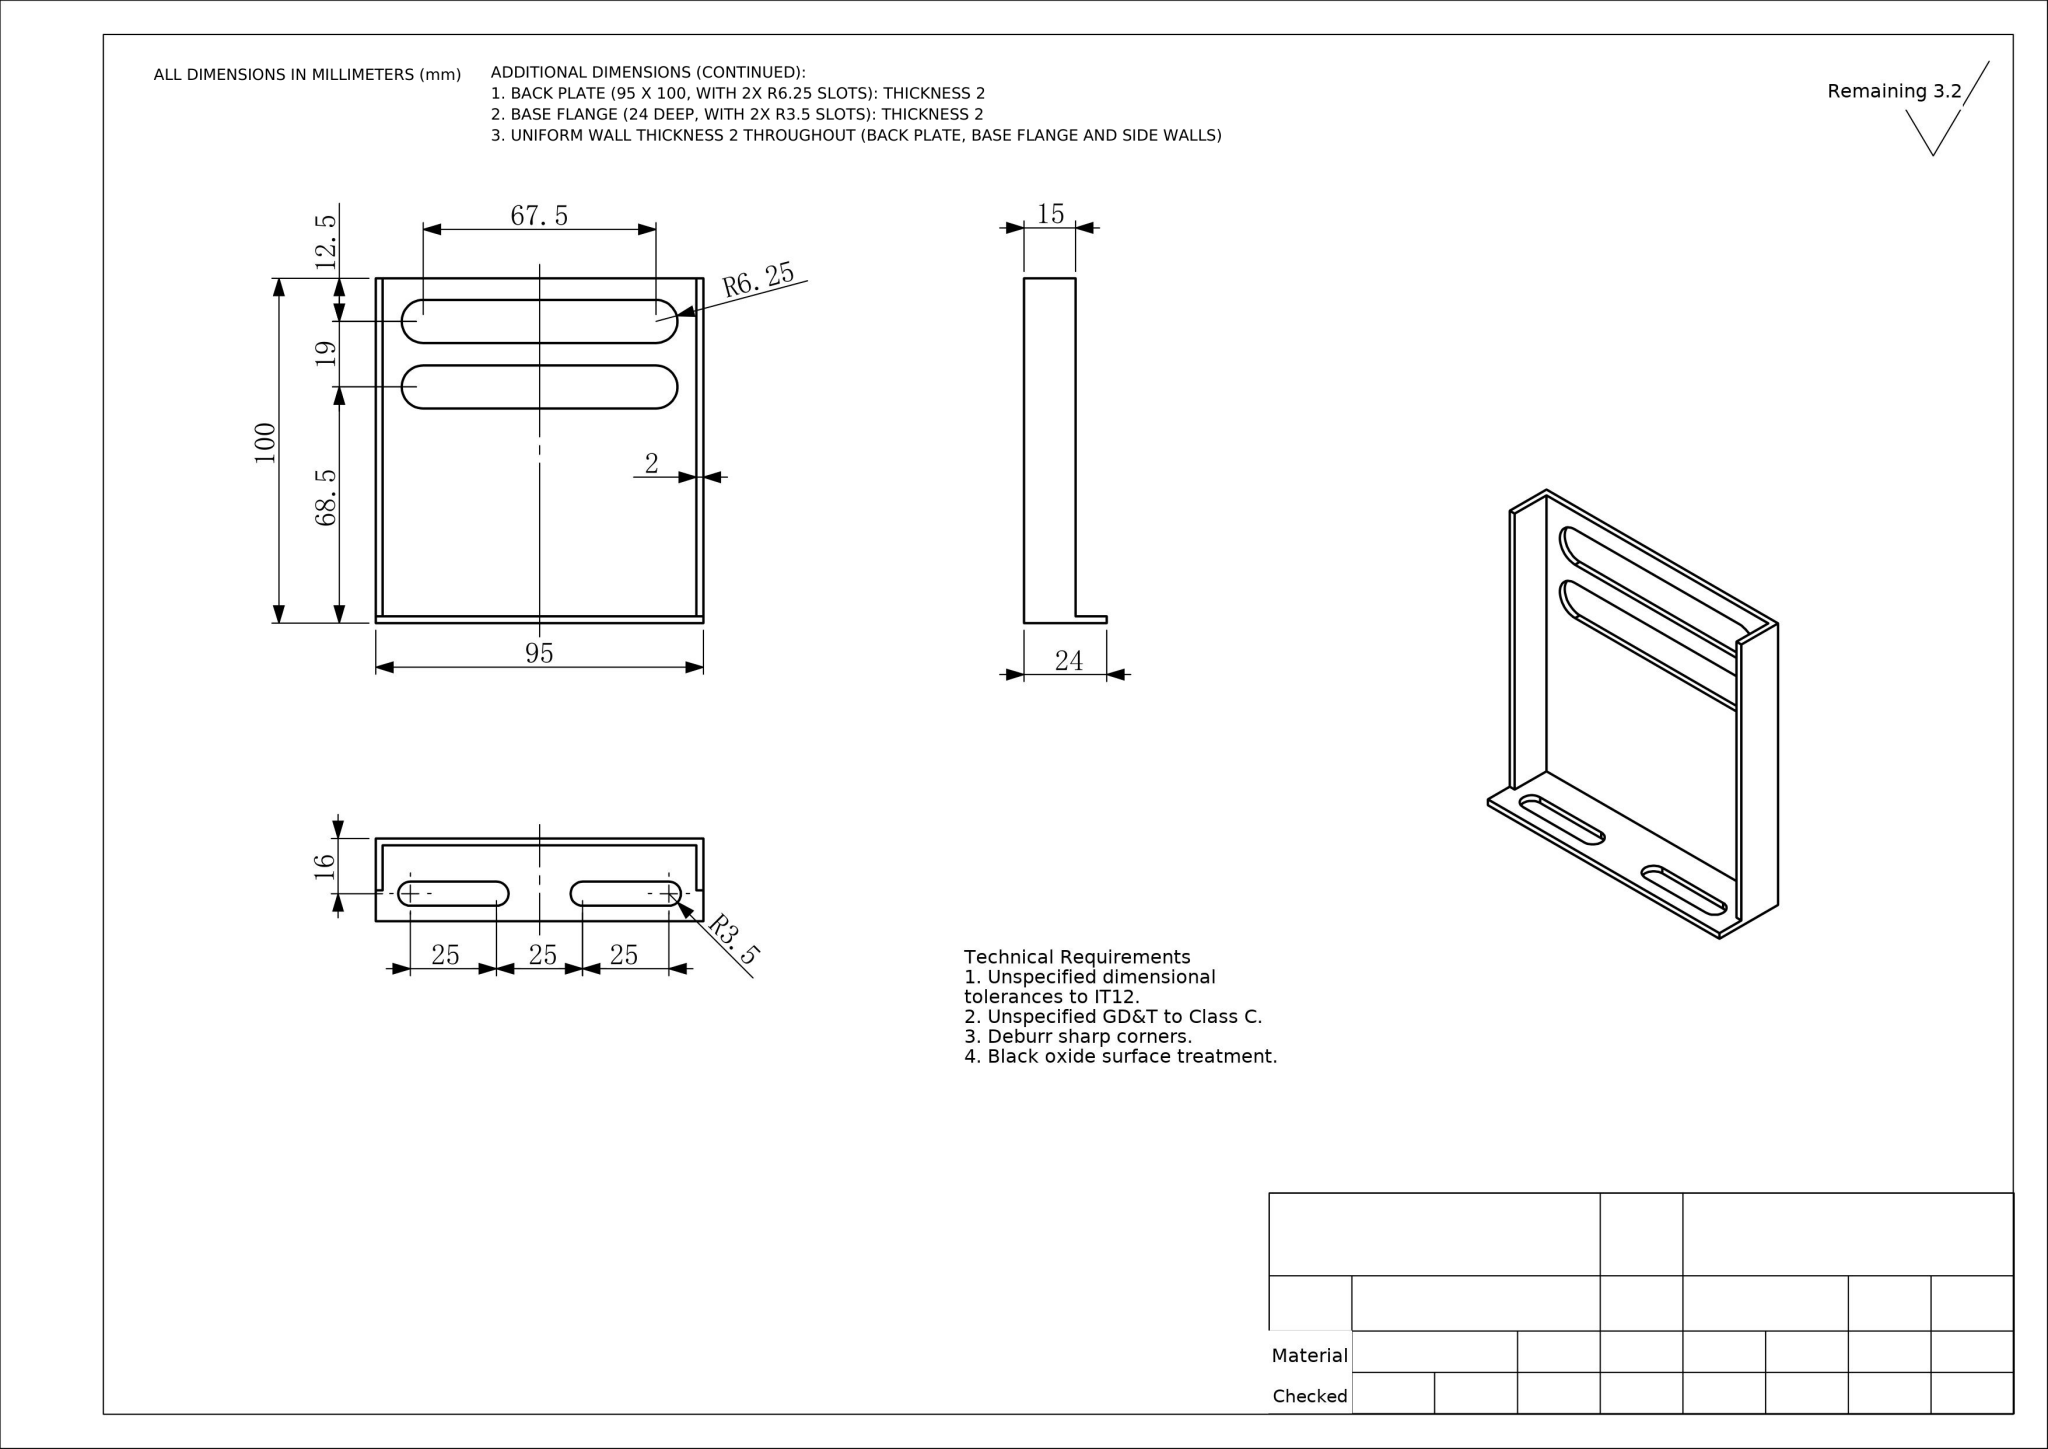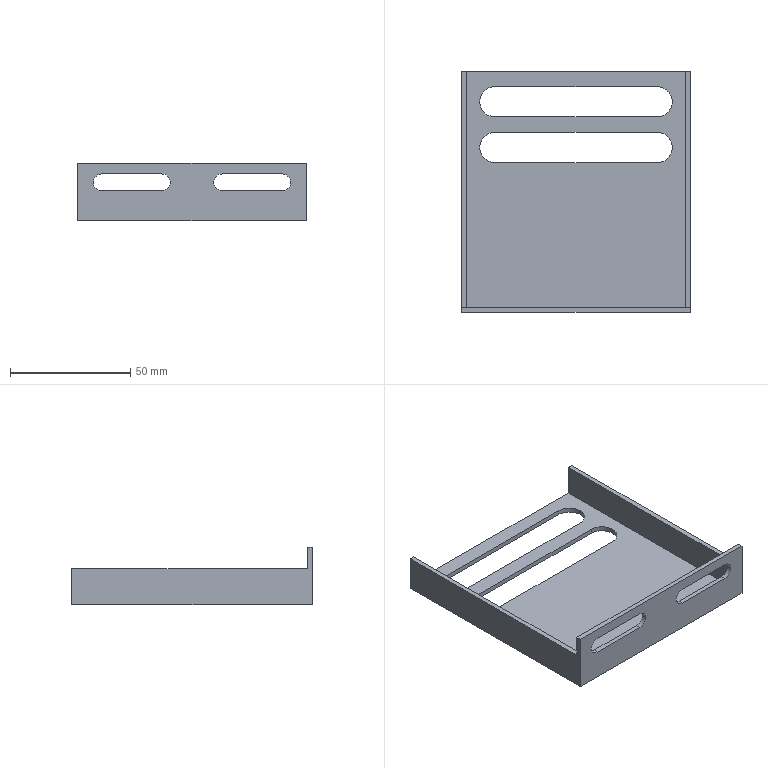Part | NX | mm | 1 solid | 30 faces | box 95 x 100 x 24 mm | volume 23556 mm3 | plane 20 | cylinder 10 | commonest cylinder face diameters 12.5 x6 7 x4
STEP:
#1=COLOUR_RGB('',0.502,0.502,1.);
#2=FILL_AREA_STYLE_COLOUR('',#1);
#3=FILL_AREA_STYLE('',(#2));
#4=SURFACE_STYLE_FILL_AREA(#3);
#5=SURFACE_SIDE_STYLE('',(#4));
#6=SURFACE_STYLE_USAGE(.BOTH.,#5);
#7=PRESENTATION_STYLE_ASSIGNMENT((#6));
#8=CARTESIAN_POINT('',(40.,87.5,0.));
#9=VERTEX_POINT('',#8);
#10=CARTESIAN_POINT('',(33.75,93.75,0.));
#11=VERTEX_POINT('',#10);
#12=CARTESIAN_POINT('',(33.75,87.5,0.));
#13=DIRECTION('',(0.,0.,1.));
#14=DIRECTION('',(-1.,0.,0.));
#15=AXIS2_PLACEMENT_3D('',#12,#13,#14);
#16=CIRCLE('',#15,6.25);
#17=EDGE_CURVE('',#9,#11,#16,.T.);
#18=ORIENTED_EDGE('',*,*,#17,.F.);
#19=CARTESIAN_POINT('',(40.,87.5,2.));
#20=VERTEX_POINT('',#19);
#21=CARTESIAN_POINT('',(40.,87.5,0.));
#22=DIRECTION('',(0.,0.,1.));
#23=VECTOR('',#22,1000.);
#24=LINE('',#21,#23);
#25=EDGE_CURVE('',#9,#20,#24,.T.);
#26=ORIENTED_EDGE('',*,*,#25,.T.);
#27=CARTESIAN_POINT('',(33.75,93.75,2.));
#28=VERTEX_POINT('',#27);
#29=CARTESIAN_POINT('',(33.75,87.5,2.));
#30=DIRECTION('',(0.,0.,1.));
#31=DIRECTION('',(-1.,0.,0.));
#32=AXIS2_PLACEMENT_3D('',#29,#30,#31);
#33=CIRCLE('',#32,6.25);
#34=EDGE_CURVE('',#20,#28,#33,.T.);
#35=ORIENTED_EDGE('',*,*,#34,.T.);
#36=CARTESIAN_POINT('',(33.75,93.75,0.));
#37=DIRECTION('',(0.,0.,1.));
#38=VECTOR('',#37,1000.);
#39=LINE('',#36,#38);
#40=EDGE_CURVE('',#11,#28,#39,.T.);
#41=ORIENTED_EDGE('',*,*,#40,.F.);
#42=EDGE_LOOP('',(#18,#26,#35,#41));
#43=FACE_OUTER_BOUND('',#42,.T.);
#44=CARTESIAN_POINT('',(33.75,87.5,0.));
#45=DIRECTION('',(0.,0.,1.));
#46=DIRECTION('',(1.,0.,0.));
#47=AXIS2_PLACEMENT_3D('',#44,#45,#46);
#48=CYLINDRICAL_SURFACE('',#47,6.25);
#49=ADVANCED_FACE('',(#43),#48,.F.);
#50=CARTESIAN_POINT('',(40.,68.5,0.));
#51=VERTEX_POINT('',#50);
#52=CARTESIAN_POINT('',(33.75,74.75,0.));
#53=VERTEX_POINT('',#52);
#54=CARTESIAN_POINT('',(33.75,68.5,0.));
#55=DIRECTION('',(0.,0.,1.));
#56=DIRECTION('',(-1.,0.,0.));
#57=AXIS2_PLACEMENT_3D('',#54,#55,#56);
#58=CIRCLE('',#57,6.25);
#59=EDGE_CURVE('',#51,#53,#58,.T.);
#60=ORIENTED_EDGE('',*,*,#59,.F.);
#61=CARTESIAN_POINT('',(40.,68.5,2.));
#62=VERTEX_POINT('',#61);
#63=CARTESIAN_POINT('',(40.,68.5,0.));
#64=DIRECTION('',(0.,0.,1.));
#65=VECTOR('',#64,1000.);
#66=LINE('',#63,#65);
#67=EDGE_CURVE('',#51,#62,#66,.T.);
#68=ORIENTED_EDGE('',*,*,#67,.T.);
#69=CARTESIAN_POINT('',(33.75,74.75,2.));
#70=VERTEX_POINT('',#69);
#71=CARTESIAN_POINT('',(33.75,68.5,2.));
#72=DIRECTION('',(0.,0.,1.));
#73=DIRECTION('',(-1.,0.,0.));
#74=AXIS2_PLACEMENT_3D('',#71,#72,#73);
#75=CIRCLE('',#74,6.25);
#76=EDGE_CURVE('',#62,#70,#75,.T.);
#77=ORIENTED_EDGE('',*,*,#76,.T.);
#78=CARTESIAN_POINT('',(33.75,74.75,0.));
#79=DIRECTION('',(0.,0.,1.));
#80=VECTOR('',#79,1000.);
#81=LINE('',#78,#80);
#82=EDGE_CURVE('',#53,#70,#81,.T.);
#83=ORIENTED_EDGE('',*,*,#82,.F.);
#84=EDGE_LOOP('',(#60,#68,#77,#83));
#85=FACE_OUTER_BOUND('',#84,.T.);
#86=CARTESIAN_POINT('',(33.75,68.5,0.));
#87=DIRECTION('',(0.,0.,1.));
#88=DIRECTION('',(1.,0.,0.));
#89=AXIS2_PLACEMENT_3D('',#86,#87,#88);
#90=CYLINDRICAL_SURFACE('',#89,6.25);
#91=ADVANCED_FACE('',(#85),#90,.F.);
#92=CARTESIAN_POINT('',(-33.75,81.25,2.));
#93=VERTEX_POINT('',#92);
#94=CARTESIAN_POINT('',(33.75,81.25,2.));
#95=VERTEX_POINT('',#94);
#96=CARTESIAN_POINT('',(-33.75,81.25,2.));
#97=DIRECTION('',(1.,-0.,0.));
#98=VECTOR('',#97,1000.);
#99=LINE('',#96,#98);
#100=EDGE_CURVE('',#93,#95,#99,.T.);
#101=ORIENTED_EDGE('',*,*,#100,.F.);
#102=CARTESIAN_POINT('',(-33.75,93.75,2.));
#103=VERTEX_POINT('',#102);
#104=CARTESIAN_POINT('',(-33.75,87.5,2.));
#105=DIRECTION('',(0.,0.,1.));
#106=DIRECTION('',(1.,0.,0.));
#107=AXIS2_PLACEMENT_3D('',#104,#105,#106);
#108=CIRCLE('',#107,6.25);
#109=EDGE_CURVE('',#103,#93,#108,.T.);
#110=ORIENTED_EDGE('',*,*,#109,.F.);
#111=CARTESIAN_POINT('',(-33.75,93.75,2.));
#112=DIRECTION('',(-1.,0.,0.));
#113=VECTOR('',#112,1000.);
#114=LINE('',#111,#113);
#115=EDGE_CURVE('',#28,#103,#114,.T.);
#116=ORIENTED_EDGE('',*,*,#115,.F.);
#117=ORIENTED_EDGE('',*,*,#34,.F.);
#118=CARTESIAN_POINT('',(33.75,87.5,2.));
#119=DIRECTION('',(0.,0.,1.));
#120=DIRECTION('',(-1.,0.,0.));
#121=AXIS2_PLACEMENT_3D('',#118,#119,#120);
#122=CIRCLE('',#121,6.25);
#123=EDGE_CURVE('',#95,#20,#122,.T.);
#124=ORIENTED_EDGE('',*,*,#123,.F.);
#125=EDGE_LOOP('',(#101,#110,#116,#117,#124));
#126=FACE_BOUND('',#125,.T.);
#127=CARTESIAN_POINT('',(-33.75,62.25,2.));
#128=VERTEX_POINT('',#127);
#129=CARTESIAN_POINT('',(33.75,62.25,2.));
#130=VERTEX_POINT('',#129);
#131=CARTESIAN_POINT('',(33.75,62.25,2.));
#132=DIRECTION('',(1.,0.,0.));
#133=VECTOR('',#132,1000.);
#134=LINE('',#131,#133);
#135=EDGE_CURVE('',#128,#130,#134,.T.);
#136=ORIENTED_EDGE('',*,*,#135,.F.);
#137=CARTESIAN_POINT('',(-33.75,74.75,2.));
#138=VERTEX_POINT('',#137);
#139=CARTESIAN_POINT('',(-33.75,68.5,2.));
#140=DIRECTION('',(0.,0.,1.));
#141=DIRECTION('',(-1.,0.,0.));
#142=AXIS2_PLACEMENT_3D('',#139,#140,#141);
#143=CIRCLE('',#142,6.25);
#144=EDGE_CURVE('',#138,#128,#143,.T.);
#145=ORIENTED_EDGE('',*,*,#144,.F.);
#146=CARTESIAN_POINT('',(-33.75,74.75,2.));
#147=DIRECTION('',(-1.,0.,0.));
#148=VECTOR('',#147,1000.);
#149=LINE('',#146,#148);
#150=EDGE_CURVE('',#70,#138,#149,.T.);
#151=ORIENTED_EDGE('',*,*,#150,.F.);
#152=ORIENTED_EDGE('',*,*,#76,.F.);
#153=CARTESIAN_POINT('',(33.75,68.5,2.));
#154=DIRECTION('',(0.,0.,1.));
#155=DIRECTION('',(-1.,0.,0.));
#156=AXIS2_PLACEMENT_3D('',#153,#154,#155);
#157=CIRCLE('',#156,6.25);
#158=EDGE_CURVE('',#130,#62,#157,.T.);
#159=ORIENTED_EDGE('',*,*,#158,.F.);
#160=EDGE_LOOP('',(#136,#145,#151,#152,#159));
#161=FACE_BOUND('',#160,.T.);
#162=CARTESIAN_POINT('',(45.5,100.,2.));
#163=VERTEX_POINT('',#162);
#164=CARTESIAN_POINT('',(45.5,2.,2.));
#165=VERTEX_POINT('',#164);
#166=CARTESIAN_POINT('',(45.5,100.,2.));
#167=DIRECTION('',(0.,-1.,-0.));
#168=VECTOR('',#167,1000.);
#169=LINE('',#166,#168);
#170=EDGE_CURVE('',#163,#165,#169,.T.);
#171=ORIENTED_EDGE('',*,*,#170,.F.);
#172=CARTESIAN_POINT('',(-45.5,100.,2.));
#173=VERTEX_POINT('',#172);
#174=CARTESIAN_POINT('',(47.5,100.,2.));
#175=DIRECTION('',(-1.,0.,0.));
#176=VECTOR('',#175,1000.);
#177=LINE('',#174,#176);
#178=EDGE_CURVE('',#163,#173,#177,.T.);
#179=ORIENTED_EDGE('',*,*,#178,.T.);
#180=CARTESIAN_POINT('',(-45.5,2.,2.));
#181=VERTEX_POINT('',#180);
#182=CARTESIAN_POINT('',(-45.5,100.,2.));
#183=DIRECTION('',(0.,1.,0.));
#184=VECTOR('',#183,1000.);
#185=LINE('',#182,#184);
#186=EDGE_CURVE('',#181,#173,#185,.T.);
#187=ORIENTED_EDGE('',*,*,#186,.F.);
#188=CARTESIAN_POINT('',(47.5,2.,2.));
#189=DIRECTION('',(-1.,0.,0.));
#190=VECTOR('',#189,1000.);
#191=LINE('',#188,#190);
#192=EDGE_CURVE('',#165,#181,#191,.T.);
#193=ORIENTED_EDGE('',*,*,#192,.F.);
#194=EDGE_LOOP('',(#171,#179,#187,#193));
#195=FACE_OUTER_BOUND('',#194,.T.);
#196=CARTESIAN_POINT('',(47.5,100.,2.));
#197=DIRECTION('',(0.,0.,-1.));
#198=DIRECTION('',(0.,1.,0.));
#199=AXIS2_PLACEMENT_3D('',#196,#197,#198);
#200=PLANE('',#199);
#201=ADVANCED_FACE('',(#126,#161,#195),#200,.F.);
#202=CARTESIAN_POINT('',(37.5,2.,12.5));
#203=VERTEX_POINT('',#202);
#204=CARTESIAN_POINT('',(12.5,2.,12.5));
#205=VERTEX_POINT('',#204);
#206=CARTESIAN_POINT('',(37.5,2.,12.5));
#207=DIRECTION('',(-1.,0.,0.));
#208=VECTOR('',#207,1000.);
#209=LINE('',#206,#208);
#210=EDGE_CURVE('',#203,#205,#209,.T.);
#211=ORIENTED_EDGE('',*,*,#210,.F.);
#212=CARTESIAN_POINT('',(37.5,2.,19.5));
#213=VERTEX_POINT('',#212);
#214=CARTESIAN_POINT('',(37.5,2.,16.));
#215=DIRECTION('',(0.,1.,0.));
#216=DIRECTION('',(0.,-0.,1.));
#217=AXIS2_PLACEMENT_3D('',#214,#215,#216);
#218=CIRCLE('',#217,3.5);
#219=EDGE_CURVE('',#213,#203,#218,.T.);
#220=ORIENTED_EDGE('',*,*,#219,.F.);
#221=CARTESIAN_POINT('',(12.5,2.,19.5));
#222=VERTEX_POINT('',#221);
#223=CARTESIAN_POINT('',(37.5,2.,19.5));
#224=DIRECTION('',(1.,0.,-0.));
#225=VECTOR('',#224,1000.);
#226=LINE('',#223,#225);
#227=EDGE_CURVE('',#222,#213,#226,.T.);
#228=ORIENTED_EDGE('',*,*,#227,.F.);
#229=CARTESIAN_POINT('',(12.5,2.,16.));
#230=DIRECTION('',(0.,1.,0.));
#231=DIRECTION('',(0.,-0.,1.));
#232=AXIS2_PLACEMENT_3D('',#229,#230,#231);
#233=CIRCLE('',#232,3.5);
#234=EDGE_CURVE('',#205,#222,#233,.T.);
#235=ORIENTED_EDGE('',*,*,#234,.F.);
#236=EDGE_LOOP('',(#211,#220,#228,#235));
#237=FACE_BOUND('',#236,.T.);
#238=CARTESIAN_POINT('',(-37.5,2.,19.5));
#239=VERTEX_POINT('',#238);
#240=CARTESIAN_POINT('',(-12.5,2.,19.5));
#241=VERTEX_POINT('',#240);
#242=CARTESIAN_POINT('',(-37.5,2.,19.5));
#243=DIRECTION('',(1.,0.,0.));
#244=VECTOR('',#243,1000.);
#245=LINE('',#242,#244);
#246=EDGE_CURVE('',#239,#241,#245,.T.);
#247=ORIENTED_EDGE('',*,*,#246,.F.);
#248=CARTESIAN_POINT('',(-37.5,2.,12.5));
#249=VERTEX_POINT('',#248);
#250=CARTESIAN_POINT('',(-37.5,2.,16.));
#251=DIRECTION('',(0.,1.,0.));
#252=DIRECTION('',(0.,-0.,1.));
#253=AXIS2_PLACEMENT_3D('',#250,#251,#252);
#254=CIRCLE('',#253,3.5);
#255=EDGE_CURVE('',#249,#239,#254,.T.);
#256=ORIENTED_EDGE('',*,*,#255,.F.);
#257=CARTESIAN_POINT('',(-12.5,2.,12.5));
#258=VERTEX_POINT('',#257);
#259=CARTESIAN_POINT('',(-37.5,2.,12.5));
#260=DIRECTION('',(-1.,0.,-0.));
#261=VECTOR('',#260,1000.);
#262=LINE('',#259,#261);
#263=EDGE_CURVE('',#258,#249,#262,.T.);
#264=ORIENTED_EDGE('',*,*,#263,.F.);
#265=CARTESIAN_POINT('',(-12.5,2.,16.));
#266=DIRECTION('',(0.,1.,0.));
#267=DIRECTION('',(0.,0.,-1.));
#268=AXIS2_PLACEMENT_3D('',#265,#266,#267);
#269=CIRCLE('',#268,3.5);
#270=EDGE_CURVE('',#241,#258,#269,.T.);
#271=ORIENTED_EDGE('',*,*,#270,.F.);
#272=EDGE_LOOP('',(#247,#256,#264,#271));
#273=FACE_BOUND('',#272,.T.);
#274=CARTESIAN_POINT('',(45.5,2.,15.));
#275=VERTEX_POINT('',#274);
#276=CARTESIAN_POINT('',(47.5,2.,15.));
#277=VERTEX_POINT('',#276);
#278=CARTESIAN_POINT('',(47.5,2.,15.));
#279=DIRECTION('',(1.,0.,0.));
#280=VECTOR('',#279,1000.);
#281=LINE('',#278,#280);
#282=EDGE_CURVE('',#275,#277,#281,.T.);
#283=ORIENTED_EDGE('',*,*,#282,.F.);
#284=CARTESIAN_POINT('',(45.5,2.,2.));
#285=DIRECTION('',(0.,-0.,1.));
#286=VECTOR('',#285,1000.);
#287=LINE('',#284,#286);
#288=EDGE_CURVE('',#165,#275,#287,.T.);
#289=ORIENTED_EDGE('',*,*,#288,.F.);
#290=ORIENTED_EDGE('',*,*,#192,.T.);
#291=CARTESIAN_POINT('',(-45.5,2.,15.));
#292=VERTEX_POINT('',#291);
#293=CARTESIAN_POINT('',(-45.5,2.,2.));
#294=DIRECTION('',(0.,0.,-1.));
#295=VECTOR('',#294,1000.);
#296=LINE('',#293,#295);
#297=EDGE_CURVE('',#292,#181,#296,.T.);
#298=ORIENTED_EDGE('',*,*,#297,.F.);
#299=CARTESIAN_POINT('',(-47.5,2.,15.));
#300=VERTEX_POINT('',#299);
#301=CARTESIAN_POINT('',(47.5,2.,15.));
#302=DIRECTION('',(-1.,0.,0.));
#303=VECTOR('',#302,1000.);
#304=LINE('',#301,#303);
#305=EDGE_CURVE('',#292,#300,#304,.T.);
#306=ORIENTED_EDGE('',*,*,#305,.T.);
#307=CARTESIAN_POINT('',(-47.5,2.,24.));
#308=VERTEX_POINT('',#307);
#309=CARTESIAN_POINT('',(-47.5,2.,2.));
#310=DIRECTION('',(0.,-0.,1.));
#311=VECTOR('',#310,1000.);
#312=LINE('',#309,#311);
#313=EDGE_CURVE('',#300,#308,#312,.T.);
#314=ORIENTED_EDGE('',*,*,#313,.T.);
#315=CARTESIAN_POINT('',(47.5,2.,24.));
#316=VERTEX_POINT('',#315);
#317=CARTESIAN_POINT('',(47.5,2.,24.));
#318=DIRECTION('',(-1.,0.,0.));
#319=VECTOR('',#318,1000.);
#320=LINE('',#317,#319);
#321=EDGE_CURVE('',#316,#308,#320,.T.);
#322=ORIENTED_EDGE('',*,*,#321,.F.);
#323=CARTESIAN_POINT('',(47.5,2.,2.));
#324=DIRECTION('',(0.,-0.,1.));
#325=VECTOR('',#324,1000.);
#326=LINE('',#323,#325);
#327=EDGE_CURVE('',#277,#316,#326,.T.);
#328=ORIENTED_EDGE('',*,*,#327,.F.);
#329=EDGE_LOOP('',(#283,#289,#290,#298,#306,#314,#322,#328));
#330=FACE_OUTER_BOUND('',#329,.T.);
#331=CARTESIAN_POINT('',(47.5,2.,2.));
#332=DIRECTION('',(0.,-1.,-0.));
#333=DIRECTION('',(0.,0.,-1.));
#334=AXIS2_PLACEMENT_3D('',#331,#332,#333);
#335=PLANE('',#334);
#336=ADVANCED_FACE('',(#237,#273,#330),#335,.F.);
#337=CARTESIAN_POINT('',(12.5,-0.,19.5));
#338=VERTEX_POINT('',#337);
#339=CARTESIAN_POINT('',(37.5,-0.,19.5));
#340=VERTEX_POINT('',#339);
#341=CARTESIAN_POINT('',(37.5,-0.,19.5));
#342=DIRECTION('',(1.,0.,-0.));
#343=VECTOR('',#342,1000.);
#344=LINE('',#341,#343);
#345=EDGE_CURVE('',#338,#340,#344,.T.);
#346=ORIENTED_EDGE('',*,*,#345,.T.);
#347=CARTESIAN_POINT('',(37.5,-0.,12.5));
#348=VERTEX_POINT('',#347);
#349=CARTESIAN_POINT('',(37.5,-0.,16.));
#350=DIRECTION('',(0.,1.,0.));
#351=DIRECTION('',(0.,-0.,1.));
#352=AXIS2_PLACEMENT_3D('',#349,#350,#351);
#353=CIRCLE('',#352,3.5);
#354=EDGE_CURVE('',#340,#348,#353,.T.);
#355=ORIENTED_EDGE('',*,*,#354,.T.);
#356=CARTESIAN_POINT('',(12.5,-0.,12.5));
#357=VERTEX_POINT('',#356);
#358=CARTESIAN_POINT('',(37.5,-0.,12.5));
#359=DIRECTION('',(-1.,0.,0.));
#360=VECTOR('',#359,1000.);
#361=LINE('',#358,#360);
#362=EDGE_CURVE('',#348,#357,#361,.T.);
#363=ORIENTED_EDGE('',*,*,#362,.T.);
#364=CARTESIAN_POINT('',(12.5,-0.,16.));
#365=DIRECTION('',(0.,1.,0.));
#366=DIRECTION('',(0.,-0.,1.));
#367=AXIS2_PLACEMENT_3D('',#364,#365,#366);
#368=CIRCLE('',#367,3.5);
#369=EDGE_CURVE('',#357,#338,#368,.T.);
#370=ORIENTED_EDGE('',*,*,#369,.T.);
#371=EDGE_LOOP('',(#346,#355,#363,#370));
#372=FACE_BOUND('',#371,.T.);
#373=CARTESIAN_POINT('',(-12.5,-0.,12.5));
#374=VERTEX_POINT('',#373);
#375=CARTESIAN_POINT('',(-37.5,-0.,12.5));
#376=VERTEX_POINT('',#375);
#377=CARTESIAN_POINT('',(-37.5,-0.,12.5));
#378=DIRECTION('',(-1.,0.,-0.));
#379=VECTOR('',#378,1000.);
#380=LINE('',#377,#379);
#381=EDGE_CURVE('',#374,#376,#380,.T.);
#382=ORIENTED_EDGE('',*,*,#381,.T.);
#383=CARTESIAN_POINT('',(-37.5,-0.,19.5));
#384=VERTEX_POINT('',#383);
#385=CARTESIAN_POINT('',(-37.5,-0.,16.));
#386=DIRECTION('',(0.,1.,0.));
#387=DIRECTION('',(0.,-0.,1.));
#388=AXIS2_PLACEMENT_3D('',#385,#386,#387);
#389=CIRCLE('',#388,3.5);
#390=EDGE_CURVE('',#376,#384,#389,.T.);
#391=ORIENTED_EDGE('',*,*,#390,.T.);
#392=CARTESIAN_POINT('',(-12.5,-0.,19.5));
#393=VERTEX_POINT('',#392);
#394=CARTESIAN_POINT('',(-37.5,-0.,19.5));
#395=DIRECTION('',(1.,0.,0.));
#396=VECTOR('',#395,1000.);
#397=LINE('',#394,#396);
#398=EDGE_CURVE('',#384,#393,#397,.T.);
#399=ORIENTED_EDGE('',*,*,#398,.T.);
#400=CARTESIAN_POINT('',(-12.5,-0.,16.));
#401=DIRECTION('',(0.,1.,0.));
#402=DIRECTION('',(0.,0.,-1.));
#403=AXIS2_PLACEMENT_3D('',#400,#401,#402);
#404=CIRCLE('',#403,3.5);
#405=EDGE_CURVE('',#393,#374,#404,.T.);
#406=ORIENTED_EDGE('',*,*,#405,.T.);
#407=EDGE_LOOP('',(#382,#391,#399,#406));
#408=FACE_BOUND('',#407,.T.);
#409=CARTESIAN_POINT('',(47.5,0.,0.));
#410=VERTEX_POINT('',#409);
#411=CARTESIAN_POINT('',(-47.5,0.,0.));
#412=VERTEX_POINT('',#411);
#413=CARTESIAN_POINT('',(47.5,0.,0.));
#414=DIRECTION('',(-1.,0.,0.));
#415=VECTOR('',#414,1000.);
#416=LINE('',#413,#415);
#417=EDGE_CURVE('',#410,#412,#416,.T.);
#418=ORIENTED_EDGE('',*,*,#417,.F.);
#419=CARTESIAN_POINT('',(47.5,-0.,24.));
#420=VERTEX_POINT('',#419);
#421=CARTESIAN_POINT('',(47.5,0.,0.));
#422=DIRECTION('',(0.,0.,-1.));
#423=VECTOR('',#422,1000.);
#424=LINE('',#421,#423);
#425=EDGE_CURVE('',#420,#410,#424,.T.);
#426=ORIENTED_EDGE('',*,*,#425,.F.);
#427=CARTESIAN_POINT('',(-47.5,-0.,24.));
#428=VERTEX_POINT('',#427);
#429=CARTESIAN_POINT('',(47.5,-0.,24.));
#430=DIRECTION('',(-1.,0.,0.));
#431=VECTOR('',#430,1000.);
#432=LINE('',#429,#431);
#433=EDGE_CURVE('',#420,#428,#432,.T.);
#434=ORIENTED_EDGE('',*,*,#433,.T.);
#435=CARTESIAN_POINT('',(-47.5,0.,0.));
#436=DIRECTION('',(0.,0.,-1.));
#437=VECTOR('',#436,1000.);
#438=LINE('',#435,#437);
#439=EDGE_CURVE('',#428,#412,#438,.T.);
#440=ORIENTED_EDGE('',*,*,#439,.T.);
#441=EDGE_LOOP('',(#418,#426,#434,#440));
#442=FACE_OUTER_BOUND('',#441,.T.);
#443=CARTESIAN_POINT('',(47.5,0.,0.));
#444=DIRECTION('',(0.,1.,0.));
#445=DIRECTION('',(0.,-0.,1.));
#446=AXIS2_PLACEMENT_3D('',#443,#444,#445);
#447=PLANE('',#446);
#448=ADVANCED_FACE('',(#372,#408,#442),#447,.F.);
#449=CARTESIAN_POINT('',(-33.75,93.75,0.));
#450=VERTEX_POINT('',#449);
#451=CARTESIAN_POINT('',(-33.75,93.75,0.));
#452=DIRECTION('',(-1.,0.,0.));
#453=VECTOR('',#452,1000.);
#454=LINE('',#451,#453);
#455=EDGE_CURVE('',#11,#450,#454,.T.);
#456=ORIENTED_EDGE('',*,*,#455,.T.);
#457=CARTESIAN_POINT('',(-33.75,81.25,0.));
#458=VERTEX_POINT('',#457);
#459=CARTESIAN_POINT('',(-33.75,87.5,0.));
#460=DIRECTION('',(0.,0.,1.));
#461=DIRECTION('',(1.,0.,0.));
#462=AXIS2_PLACEMENT_3D('',#459,#460,#461);
#463=CIRCLE('',#462,6.25);
#464=EDGE_CURVE('',#450,#458,#463,.T.);
#465=ORIENTED_EDGE('',*,*,#464,.T.);
#466=CARTESIAN_POINT('',(33.75,81.25,0.));
#467=VERTEX_POINT('',#466);
#468=CARTESIAN_POINT('',(-33.75,81.25,0.));
#469=DIRECTION('',(1.,-0.,0.));
#470=VECTOR('',#469,1000.);
#471=LINE('',#468,#470);
#472=EDGE_CURVE('',#458,#467,#471,.T.);
#473=ORIENTED_EDGE('',*,*,#472,.T.);
#474=CARTESIAN_POINT('',(33.75,87.5,0.));
#475=DIRECTION('',(0.,0.,1.));
#476=DIRECTION('',(-1.,0.,0.));
#477=AXIS2_PLACEMENT_3D('',#474,#475,#476);
#478=CIRCLE('',#477,6.25);
#479=EDGE_CURVE('',#467,#9,#478,.T.);
#480=ORIENTED_EDGE('',*,*,#479,.T.);
#481=ORIENTED_EDGE('',*,*,#17,.T.);
#482=EDGE_LOOP('',(#456,#465,#473,#480,#481));
#483=FACE_BOUND('',#482,.T.);
#484=CARTESIAN_POINT('',(-33.75,74.75,0.));
#485=VERTEX_POINT('',#484);
#486=CARTESIAN_POINT('',(-33.75,74.75,0.));
#487=DIRECTION('',(-1.,0.,0.));
#488=VECTOR('',#487,1000.);
#489=LINE('',#486,#488);
#490=EDGE_CURVE('',#53,#485,#489,.T.);
#491=ORIENTED_EDGE('',*,*,#490,.T.);
#492=CARTESIAN_POINT('',(-33.75,62.25,0.));
#493=VERTEX_POINT('',#492);
#494=CARTESIAN_POINT('',(-33.75,68.5,0.));
#495=DIRECTION('',(0.,0.,1.));
#496=DIRECTION('',(-1.,0.,0.));
#497=AXIS2_PLACEMENT_3D('',#494,#495,#496);
#498=CIRCLE('',#497,6.25);
#499=EDGE_CURVE('',#485,#493,#498,.T.);
#500=ORIENTED_EDGE('',*,*,#499,.T.);
#501=CARTESIAN_POINT('',(33.75,62.25,0.));
#502=VERTEX_POINT('',#501);
#503=CARTESIAN_POINT('',(33.75,62.25,0.));
#504=DIRECTION('',(1.,0.,0.));
#505=VECTOR('',#504,1000.);
#506=LINE('',#503,#505);
#507=EDGE_CURVE('',#493,#502,#506,.T.);
#508=ORIENTED_EDGE('',*,*,#507,.T.);
#509=CARTESIAN_POINT('',(33.75,68.5,0.));
#510=DIRECTION('',(0.,0.,1.));
#511=DIRECTION('',(-1.,0.,0.));
#512=AXIS2_PLACEMENT_3D('',#509,#510,#511);
#513=CIRCLE('',#512,6.25);
#514=EDGE_CURVE('',#502,#51,#513,.T.);
#515=ORIENTED_EDGE('',*,*,#514,.T.);
#516=ORIENTED_EDGE('',*,*,#59,.T.);
#517=EDGE_LOOP('',(#491,#500,#508,#515,#516));
#518=FACE_BOUND('',#517,.T.);
#519=ORIENTED_EDGE('',*,*,#417,.T.);
#520=CARTESIAN_POINT('',(-47.5,100.,0.));
#521=VERTEX_POINT('',#520);
#522=CARTESIAN_POINT('',(-47.5,0.,0.));
#523=DIRECTION('',(0.,1.,0.));
#524=VECTOR('',#523,1000.);
#525=LINE('',#522,#524);
#526=EDGE_CURVE('',#412,#521,#525,.T.);
#527=ORIENTED_EDGE('',*,*,#526,.T.);
#528=CARTESIAN_POINT('',(47.5,100.,0.));
#529=VERTEX_POINT('',#528);
#530=CARTESIAN_POINT('',(47.5,100.,0.));
#531=DIRECTION('',(-1.,0.,0.));
#532=VECTOR('',#531,1000.);
#533=LINE('',#530,#532);
#534=EDGE_CURVE('',#529,#521,#533,.T.);
#535=ORIENTED_EDGE('',*,*,#534,.F.);
#536=CARTESIAN_POINT('',(47.5,0.,0.));
#537=DIRECTION('',(0.,1.,0.));
#538=VECTOR('',#537,1000.);
#539=LINE('',#536,#538);
#540=EDGE_CURVE('',#410,#529,#539,.T.);
#541=ORIENTED_EDGE('',*,*,#540,.F.);
#542=EDGE_LOOP('',(#519,#527,#535,#541));
#543=FACE_OUTER_BOUND('',#542,.T.);
#544=CARTESIAN_POINT('',(47.5,0.,0.));
#545=DIRECTION('',(0.,0.,1.));
#546=DIRECTION('',(1.,0.,0.));
#547=AXIS2_PLACEMENT_3D('',#544,#545,#546);
#548=PLANE('',#547);
#549=ADVANCED_FACE('',(#483,#518,#543),#548,.F.);
#550=ORIENTED_EDGE('',*,*,#534,.T.);
#551=CARTESIAN_POINT('',(-47.5,100.,15.));
#552=VERTEX_POINT('',#551);
#553=CARTESIAN_POINT('',(-47.5,100.,0.));
#554=DIRECTION('',(0.,0.,1.));
#555=VECTOR('',#554,1000.);
#556=LINE('',#553,#555);
#557=EDGE_CURVE('',#521,#552,#556,.T.);
#558=ORIENTED_EDGE('',*,*,#557,.T.);
#559=CARTESIAN_POINT('',(-45.5,100.,15.));
#560=VERTEX_POINT('',#559);
#561=CARTESIAN_POINT('',(-45.5,100.,15.));
#562=DIRECTION('',(-1.,0.,0.));
#563=VECTOR('',#562,1000.);
#564=LINE('',#561,#563);
#565=EDGE_CURVE('',#560,#552,#564,.T.);
#566=ORIENTED_EDGE('',*,*,#565,.F.);
#567=CARTESIAN_POINT('',(-45.5,100.,0.));
#568=DIRECTION('',(0.,0.,-1.));
#569=VECTOR('',#568,1000.);
#570=LINE('',#567,#569);
#571=EDGE_CURVE('',#560,#173,#570,.T.);
#572=ORIENTED_EDGE('',*,*,#571,.T.);
#573=ORIENTED_EDGE('',*,*,#178,.F.);
#574=CARTESIAN_POINT('',(45.5,100.,15.));
#575=VERTEX_POINT('',#574);
#576=CARTESIAN_POINT('',(45.5,100.,0.));
#577=DIRECTION('',(0.,0.,-1.));
#578=VECTOR('',#577,1000.);
#579=LINE('',#576,#578);
#580=EDGE_CURVE('',#575,#163,#579,.T.);
#581=ORIENTED_EDGE('',*,*,#580,.F.);
#582=CARTESIAN_POINT('',(47.5,100.,15.));
#583=VERTEX_POINT('',#582);
#584=CARTESIAN_POINT('',(45.5,100.,15.));
#585=DIRECTION('',(1.,0.,0.));
#586=VECTOR('',#585,1000.);
#587=LINE('',#584,#586);
#588=EDGE_CURVE('',#575,#583,#587,.T.);
#589=ORIENTED_EDGE('',*,*,#588,.T.);
#590=CARTESIAN_POINT('',(47.5,100.,0.));
#591=DIRECTION('',(0.,0.,1.));
#592=VECTOR('',#591,1000.);
#593=LINE('',#590,#592);
#594=EDGE_CURVE('',#529,#583,#593,.T.);
#595=ORIENTED_EDGE('',*,*,#594,.F.);
#596=EDGE_LOOP('',(#550,#558,#566,#572,#573,#581,#589,#595));
#597=FACE_OUTER_BOUND('',#596,.T.);
#598=CARTESIAN_POINT('',(47.5,100.,0.));
#599=DIRECTION('',(0.,-1.,0.));
#600=DIRECTION('',(0.,0.,-1.));
#601=AXIS2_PLACEMENT_3D('',#598,#599,#600);
#602=PLANE('',#601);
#603=ADVANCED_FACE('',(#597),#602,.F.);
#604=CARTESIAN_POINT('',(-47.5,2.,24.));
#605=DIRECTION('',(0.,-1.,0.));
#606=VECTOR('',#605,1000.);
#607=LINE('',#604,#606);
#608=EDGE_CURVE('',#308,#428,#607,.T.);
#609=ORIENTED_EDGE('',*,*,#608,.T.);
#610=ORIENTED_EDGE('',*,*,#433,.F.);
#611=CARTESIAN_POINT('',(47.5,2.,24.));
#612=DIRECTION('',(0.,-1.,0.));
#613=VECTOR('',#612,1000.);
#614=LINE('',#611,#613);
#615=EDGE_CURVE('',#316,#420,#614,.T.);
#616=ORIENTED_EDGE('',*,*,#615,.F.);
#617=ORIENTED_EDGE('',*,*,#321,.T.);
#618=EDGE_LOOP('',(#609,#610,#616,#617));
#619=FACE_OUTER_BOUND('',#618,.T.);
#620=CARTESIAN_POINT('',(47.5,2.,24.));
#621=DIRECTION('',(0.,0.,-1.));
#622=DIRECTION('',(-1.,0.,0.));
#623=AXIS2_PLACEMENT_3D('',#620,#621,#622);
#624=PLANE('',#623);
#625=ADVANCED_FACE('',(#619),#624,.F.);
#626=ORIENTED_EDGE('',*,*,#594,.T.);
#627=CARTESIAN_POINT('',(47.5,100.,15.));
#628=DIRECTION('',(0.,1.,-0.));
#629=VECTOR('',#628,1000.);
#630=LINE('',#627,#629);
#631=EDGE_CURVE('',#277,#583,#630,.T.);
#632=ORIENTED_EDGE('',*,*,#631,.F.);
#633=ORIENTED_EDGE('',*,*,#327,.T.);
#634=ORIENTED_EDGE('',*,*,#615,.T.);
#635=ORIENTED_EDGE('',*,*,#425,.T.);
#636=ORIENTED_EDGE('',*,*,#540,.T.);
#637=EDGE_LOOP('',(#626,#632,#633,#634,#635,#636));
#638=FACE_OUTER_BOUND('',#637,.T.);
#639=CARTESIAN_POINT('',(47.5,-0.,24.));
#640=DIRECTION('',(1.,0.,0.));
#641=DIRECTION('',(0.,0.,-1.));
#642=AXIS2_PLACEMENT_3D('',#639,#640,#641);
#643=PLANE('',#642);
#644=ADVANCED_FACE('',(#638),#643,.T.);
#645=ORIENTED_EDGE('',*,*,#313,.F.);
#646=CARTESIAN_POINT('',(-47.5,100.,15.));
#647=DIRECTION('',(0.,1.,-0.));
#648=VECTOR('',#647,1000.);
#649=LINE('',#646,#648);
#650=EDGE_CURVE('',#300,#552,#649,.T.);
#651=ORIENTED_EDGE('',*,*,#650,.T.);
#652=ORIENTED_EDGE('',*,*,#557,.F.);
#653=ORIENTED_EDGE('',*,*,#526,.F.);
#654=ORIENTED_EDGE('',*,*,#439,.F.);
#655=ORIENTED_EDGE('',*,*,#608,.F.);
#656=EDGE_LOOP('',(#645,#651,#652,#653,#654,#655));
#657=FACE_OUTER_BOUND('',#656,.T.);
#658=CARTESIAN_POINT('',(-47.5,-0.,24.));
#659=DIRECTION('',(1.,0.,0.));
#660=DIRECTION('',(0.,0.,-1.));
#661=AXIS2_PLACEMENT_3D('',#658,#659,#660);
#662=PLANE('',#661);
#663=ADVANCED_FACE('',(#657),#662,.F.);
#664=ORIENTED_EDGE('',*,*,#297,.T.);
#665=ORIENTED_EDGE('',*,*,#186,.T.);
#666=ORIENTED_EDGE('',*,*,#571,.F.);
#667=CARTESIAN_POINT('',(-45.5,100.,15.));
#668=DIRECTION('',(0.,1.,-0.));
#669=VECTOR('',#668,1000.);
#670=LINE('',#667,#669);
#671=EDGE_CURVE('',#292,#560,#670,.T.);
#672=ORIENTED_EDGE('',*,*,#671,.F.);
#673=EDGE_LOOP('',(#664,#665,#666,#672));
#674=FACE_OUTER_BOUND('',#673,.T.);
#675=CARTESIAN_POINT('',(-45.5,-0.,-0.));
#676=DIRECTION('',(-1.,0.,0.));
#677=DIRECTION('',(0.,0.,1.));
#678=AXIS2_PLACEMENT_3D('',#675,#676,#677);
#679=PLANE('',#678);
#680=ADVANCED_FACE('',(#674),#679,.F.);
#681=ORIENTED_EDGE('',*,*,#305,.F.);
#682=ORIENTED_EDGE('',*,*,#671,.T.);
#683=ORIENTED_EDGE('',*,*,#565,.T.);
#684=ORIENTED_EDGE('',*,*,#650,.F.);
#685=EDGE_LOOP('',(#681,#682,#683,#684));
#686=FACE_OUTER_BOUND('',#685,.T.);
#687=CARTESIAN_POINT('',(-45.5,100.,15.));
#688=DIRECTION('',(0.,0.,1.));
#689=DIRECTION('',(0.,-1.,0.));
#690=AXIS2_PLACEMENT_3D('',#687,#688,#689);
#691=PLANE('',#690);
#692=ADVANCED_FACE('',(#686),#691,.T.);
#693=ORIENTED_EDGE('',*,*,#580,.T.);
#694=ORIENTED_EDGE('',*,*,#170,.T.);
#695=ORIENTED_EDGE('',*,*,#288,.T.);
#696=CARTESIAN_POINT('',(45.5,100.,15.));
#697=DIRECTION('',(0.,1.,-0.));
#698=VECTOR('',#697,1000.);
#699=LINE('',#696,#698);
#700=EDGE_CURVE('',#275,#575,#699,.T.);
#701=ORIENTED_EDGE('',*,*,#700,.T.);
#702=EDGE_LOOP('',(#693,#694,#695,#701));
#703=FACE_OUTER_BOUND('',#702,.T.);
#704=CARTESIAN_POINT('',(45.5,-0.,-0.));
#705=DIRECTION('',(1.,0.,0.));
#706=DIRECTION('',(0.,0.,1.));
#707=AXIS2_PLACEMENT_3D('',#704,#705,#706);
#708=PLANE('',#707);
#709=ADVANCED_FACE('',(#703),#708,.F.);
#710=ORIENTED_EDGE('',*,*,#700,.F.);
#711=ORIENTED_EDGE('',*,*,#282,.T.);
#712=ORIENTED_EDGE('',*,*,#631,.T.);
#713=ORIENTED_EDGE('',*,*,#588,.F.);
#714=EDGE_LOOP('',(#710,#711,#712,#713));
#715=FACE_OUTER_BOUND('',#714,.T.);
#716=CARTESIAN_POINT('',(45.5,100.,15.));
#717=DIRECTION('',(0.,-0.,-1.));
#718=DIRECTION('',(0.,1.,-0.));
#719=AXIS2_PLACEMENT_3D('',#716,#717,#718);
#720=PLANE('',#719);
#721=ADVANCED_FACE('',(#715),#720,.F.);
#722=ORIENTED_EDGE('',*,*,#255,.T.);
#723=CARTESIAN_POINT('',(-37.5,-0.,19.5));
#724=DIRECTION('',(0.,1.,0.));
#725=VECTOR('',#724,1000.);
#726=LINE('',#723,#725);
#727=EDGE_CURVE('',#384,#239,#726,.T.);
#728=ORIENTED_EDGE('',*,*,#727,.F.);
#729=ORIENTED_EDGE('',*,*,#390,.F.);
#730=CARTESIAN_POINT('',(-37.5,-0.,12.5));
#731=DIRECTION('',(0.,1.,0.));
#732=VECTOR('',#731,1000.);
#733=LINE('',#730,#732);
#734=EDGE_CURVE('',#376,#249,#733,.T.);
#735=ORIENTED_EDGE('',*,*,#734,.T.);
#736=EDGE_LOOP('',(#722,#728,#729,#735));
#737=FACE_OUTER_BOUND('',#736,.T.);
#738=CARTESIAN_POINT('',(-37.5,-0.,16.));
#739=DIRECTION('',(0.,1.,0.));
#740=DIRECTION('',(0.,-0.,1.));
#741=AXIS2_PLACEMENT_3D('',#738,#739,#740);
#742=CYLINDRICAL_SURFACE('',#741,3.5);
#743=ADVANCED_FACE('',(#737),#742,.F.);
#744=ORIENTED_EDGE('',*,*,#263,.T.);
#745=ORIENTED_EDGE('',*,*,#734,.F.);
#746=ORIENTED_EDGE('',*,*,#381,.F.);
#747=CARTESIAN_POINT('',(-12.5,-0.,12.5));
#748=DIRECTION('',(0.,1.,0.));
#749=VECTOR('',#748,1000.);
#750=LINE('',#747,#749);
#751=EDGE_CURVE('',#374,#258,#750,.T.);
#752=ORIENTED_EDGE('',*,*,#751,.T.);
#753=EDGE_LOOP('',(#744,#745,#746,#752));
#754=FACE_OUTER_BOUND('',#753,.T.);
#755=CARTESIAN_POINT('',(-37.5,-0.,12.5));
#756=DIRECTION('',(0.,0.,-1.));
#757=DIRECTION('',(-1.,0.,-0.));
#758=AXIS2_PLACEMENT_3D('',#755,#756,#757);
#759=PLANE('',#758);
#760=ADVANCED_FACE('',(#754),#759,.F.);
#761=ORIENTED_EDGE('',*,*,#270,.T.);
#762=ORIENTED_EDGE('',*,*,#751,.F.);
#763=ORIENTED_EDGE('',*,*,#405,.F.);
#764=CARTESIAN_POINT('',(-12.5,-0.,19.5));
#765=DIRECTION('',(0.,1.,0.));
#766=VECTOR('',#765,1000.);
#767=LINE('',#764,#766);
#768=EDGE_CURVE('',#393,#241,#767,.T.);
#769=ORIENTED_EDGE('',*,*,#768,.T.);
#770=EDGE_LOOP('',(#761,#762,#763,#769));
#771=FACE_OUTER_BOUND('',#770,.T.);
#772=CARTESIAN_POINT('',(-12.5,-0.,16.));
#773=DIRECTION('',(0.,1.,0.));
#774=DIRECTION('',(0.,-0.,1.));
#775=AXIS2_PLACEMENT_3D('',#772,#773,#774);
#776=CYLINDRICAL_SURFACE('',#775,3.5);
#777=ADVANCED_FACE('',(#771),#776,.F.);
#778=ORIENTED_EDGE('',*,*,#246,.T.);
#779=ORIENTED_EDGE('',*,*,#768,.F.);
#780=ORIENTED_EDGE('',*,*,#398,.F.);
#781=ORIENTED_EDGE('',*,*,#727,.T.);
#782=EDGE_LOOP('',(#778,#779,#780,#781));
#783=FACE_OUTER_BOUND('',#782,.T.);
#784=CARTESIAN_POINT('',(-37.5,-0.,19.5));
#785=DIRECTION('',(-0.,-0.,1.));
#786=DIRECTION('',(1.,0.,0.));
#787=AXIS2_PLACEMENT_3D('',#784,#785,#786);
#788=PLANE('',#787);
#789=ADVANCED_FACE('',(#783),#788,.F.);
#790=ORIENTED_EDGE('',*,*,#219,.T.);
#791=CARTESIAN_POINT('',(37.5,-0.,12.5));
#792=DIRECTION('',(0.,1.,0.));
#793=VECTOR('',#792,1000.);
#794=LINE('',#791,#793);
#795=EDGE_CURVE('',#348,#203,#794,.T.);
#796=ORIENTED_EDGE('',*,*,#795,.F.);
#797=ORIENTED_EDGE('',*,*,#354,.F.);
#798=CARTESIAN_POINT('',(37.5,-0.,19.5));
#799=DIRECTION('',(0.,1.,0.));
#800=VECTOR('',#799,1000.);
#801=LINE('',#798,#800);
#802=EDGE_CURVE('',#340,#213,#801,.T.);
#803=ORIENTED_EDGE('',*,*,#802,.T.);
#804=EDGE_LOOP('',(#790,#796,#797,#803));
#805=FACE_OUTER_BOUND('',#804,.T.);
#806=CARTESIAN_POINT('',(37.5,-0.,16.));
#807=DIRECTION('',(0.,1.,0.));
#808=DIRECTION('',(0.,-0.,1.));
#809=AXIS2_PLACEMENT_3D('',#806,#807,#808);
#810=CYLINDRICAL_SURFACE('',#809,3.5);
#811=ADVANCED_FACE('',(#805),#810,.F.);
#812=ORIENTED_EDGE('',*,*,#227,.T.);
#813=ORIENTED_EDGE('',*,*,#802,.F.);
#814=ORIENTED_EDGE('',*,*,#345,.F.);
#815=CARTESIAN_POINT('',(12.5,-0.,19.5));
#816=DIRECTION('',(0.,1.,0.));
#817=VECTOR('',#816,1000.);
#818=LINE('',#815,#817);
#819=EDGE_CURVE('',#338,#222,#818,.T.);
#820=ORIENTED_EDGE('',*,*,#819,.T.);
#821=EDGE_LOOP('',(#812,#813,#814,#820));
#822=FACE_OUTER_BOUND('',#821,.T.);
#823=CARTESIAN_POINT('',(37.5,-0.,19.5));
#824=DIRECTION('',(0.,-0.,1.));
#825=DIRECTION('',(1.,0.,-0.));
#826=AXIS2_PLACEMENT_3D('',#823,#824,#825);
#827=PLANE('',#826);
#828=ADVANCED_FACE('',(#822),#827,.F.);
#829=ORIENTED_EDGE('',*,*,#234,.T.);
#830=ORIENTED_EDGE('',*,*,#819,.F.);
#831=ORIENTED_EDGE('',*,*,#369,.F.);
#832=CARTESIAN_POINT('',(12.5,-0.,12.5));
#833=DIRECTION('',(0.,1.,0.));
#834=VECTOR('',#833,1000.);
#835=LINE('',#832,#834);
#836=EDGE_CURVE('',#357,#205,#835,.T.);
#837=ORIENTED_EDGE('',*,*,#836,.T.);
#838=EDGE_LOOP('',(#829,#830,#831,#837));
#839=FACE_OUTER_BOUND('',#838,.T.);
#840=CARTESIAN_POINT('',(12.5,-0.,16.));
#841=DIRECTION('',(0.,1.,0.));
#842=DIRECTION('',(0.,-0.,1.));
#843=AXIS2_PLACEMENT_3D('',#840,#841,#842);
#844=CYLINDRICAL_SURFACE('',#843,3.5);
#845=ADVANCED_FACE('',(#839),#844,.F.);
#846=ORIENTED_EDGE('',*,*,#210,.T.);
#847=ORIENTED_EDGE('',*,*,#836,.F.);
#848=ORIENTED_EDGE('',*,*,#362,.F.);
#849=ORIENTED_EDGE('',*,*,#795,.T.);
#850=EDGE_LOOP('',(#846,#847,#848,#849));
#851=FACE_OUTER_BOUND('',#850,.T.);
#852=CARTESIAN_POINT('',(37.5,-0.,12.5));
#853=DIRECTION('',(-0.,0.,-1.));
#854=DIRECTION('',(0.,1.,0.));
#855=AXIS2_PLACEMENT_3D('',#852,#853,#854);
#856=PLANE('',#855);
#857=ADVANCED_FACE('',(#851),#856,.F.);
#858=ORIENTED_EDGE('',*,*,#144,.T.);
#859=CARTESIAN_POINT('',(-33.75,62.25,0.));
#860=DIRECTION('',(0.,0.,1.));
#861=VECTOR('',#860,1000.);
#862=LINE('',#859,#861);
#863=EDGE_CURVE('',#493,#128,#862,.T.);
#864=ORIENTED_EDGE('',*,*,#863,.F.);
#865=ORIENTED_EDGE('',*,*,#499,.F.);
#866=CARTESIAN_POINT('',(-33.75,74.75,0.));
#867=DIRECTION('',(0.,0.,1.));
#868=VECTOR('',#867,1000.);
#869=LINE('',#866,#868);
#870=EDGE_CURVE('',#485,#138,#869,.T.);
#871=ORIENTED_EDGE('',*,*,#870,.T.);
#872=EDGE_LOOP('',(#858,#864,#865,#871));
#873=FACE_OUTER_BOUND('',#872,.T.);
#874=CARTESIAN_POINT('',(-33.75,68.5,0.));
#875=DIRECTION('',(0.,0.,1.));
#876=DIRECTION('',(1.,0.,0.));
#877=AXIS2_PLACEMENT_3D('',#874,#875,#876);
#878=CYLINDRICAL_SURFACE('',#877,6.25);
#879=ADVANCED_FACE('',(#873),#878,.F.);
#880=ORIENTED_EDGE('',*,*,#150,.T.);
#881=ORIENTED_EDGE('',*,*,#870,.F.);
#882=ORIENTED_EDGE('',*,*,#490,.F.);
#883=ORIENTED_EDGE('',*,*,#82,.T.);
#884=EDGE_LOOP('',(#880,#881,#882,#883));
#885=FACE_OUTER_BOUND('',#884,.T.);
#886=CARTESIAN_POINT('',(-33.75,74.75,0.));
#887=DIRECTION('',(0.,1.,0.));
#888=DIRECTION('',(0.,0.,1.));
#889=AXIS2_PLACEMENT_3D('',#886,#887,#888);
#890=PLANE('',#889);
#891=ADVANCED_FACE('',(#885),#890,.F.);
#892=ORIENTED_EDGE('',*,*,#67,.F.);
#893=ORIENTED_EDGE('',*,*,#514,.F.);
#894=CARTESIAN_POINT('',(33.75,62.25,0.));
#895=DIRECTION('',(0.,0.,1.));
#896=VECTOR('',#895,1000.);
#897=LINE('',#894,#896);
#898=EDGE_CURVE('',#502,#130,#897,.T.);
#899=ORIENTED_EDGE('',*,*,#898,.T.);
#900=ORIENTED_EDGE('',*,*,#158,.T.);
#901=EDGE_LOOP('',(#892,#893,#899,#900));
#902=FACE_OUTER_BOUND('',#901,.T.);
#903=CARTESIAN_POINT('',(33.75,68.5,0.));
#904=DIRECTION('',(0.,0.,1.));
#905=DIRECTION('',(1.,0.,0.));
#906=AXIS2_PLACEMENT_3D('',#903,#904,#905);
#907=CYLINDRICAL_SURFACE('',#906,6.25);
#908=ADVANCED_FACE('',(#902),#907,.F.);
#909=ORIENTED_EDGE('',*,*,#135,.T.);
#910=ORIENTED_EDGE('',*,*,#898,.F.);
#911=ORIENTED_EDGE('',*,*,#507,.F.);
#912=ORIENTED_EDGE('',*,*,#863,.T.);
#913=EDGE_LOOP('',(#909,#910,#911,#912));
#914=FACE_OUTER_BOUND('',#913,.T.);
#915=CARTESIAN_POINT('',(33.75,62.25,0.));
#916=DIRECTION('',(0.,-1.,0.));
#917=DIRECTION('',(0.,0.,-1.));
#918=AXIS2_PLACEMENT_3D('',#915,#916,#917);
#919=PLANE('',#918);
#920=ADVANCED_FACE('',(#914),#919,.F.);
#921=ORIENTED_EDGE('',*,*,#109,.T.);
#922=CARTESIAN_POINT('',(-33.75,81.25,0.));
#923=DIRECTION('',(0.,0.,1.));
#924=VECTOR('',#923,1000.);
#925=LINE('',#922,#924);
#926=EDGE_CURVE('',#458,#93,#925,.T.);
#927=ORIENTED_EDGE('',*,*,#926,.F.);
#928=ORIENTED_EDGE('',*,*,#464,.F.);
#929=CARTESIAN_POINT('',(-33.75,93.75,0.));
#930=DIRECTION('',(0.,0.,1.));
#931=VECTOR('',#930,1000.);
#932=LINE('',#929,#931);
#933=EDGE_CURVE('',#450,#103,#932,.T.);
#934=ORIENTED_EDGE('',*,*,#933,.T.);
#935=EDGE_LOOP('',(#921,#927,#928,#934));
#936=FACE_OUTER_BOUND('',#935,.T.);
#937=CARTESIAN_POINT('',(-33.75,87.5,0.));
#938=DIRECTION('',(0.,0.,1.));
#939=DIRECTION('',(1.,0.,0.));
#940=AXIS2_PLACEMENT_3D('',#937,#938,#939);
#941=CYLINDRICAL_SURFACE('',#940,6.25);
#942=ADVANCED_FACE('',(#936),#941,.F.);
#943=ORIENTED_EDGE('',*,*,#115,.T.);
#944=ORIENTED_EDGE('',*,*,#933,.F.);
#945=ORIENTED_EDGE('',*,*,#455,.F.);
#946=ORIENTED_EDGE('',*,*,#40,.T.);
#947=EDGE_LOOP('',(#943,#944,#945,#946));
#948=FACE_OUTER_BOUND('',#947,.T.);
#949=CARTESIAN_POINT('',(-33.75,93.75,0.));
#950=DIRECTION('',(0.,1.,0.));
#951=DIRECTION('',(0.,0.,1.));
#952=AXIS2_PLACEMENT_3D('',#949,#950,#951);
#953=PLANE('',#952);
#954=ADVANCED_FACE('',(#948),#953,.F.);
#955=ORIENTED_EDGE('',*,*,#25,.F.);
#956=ORIENTED_EDGE('',*,*,#479,.F.);
#957=CARTESIAN_POINT('',(33.75,81.25,0.));
#958=DIRECTION('',(0.,0.,1.));
#959=VECTOR('',#958,1000.);
#960=LINE('',#957,#959);
#961=EDGE_CURVE('',#467,#95,#960,.T.);
#962=ORIENTED_EDGE('',*,*,#961,.T.);
#963=ORIENTED_EDGE('',*,*,#123,.T.);
#964=EDGE_LOOP('',(#955,#956,#962,#963));
#965=FACE_OUTER_BOUND('',#964,.T.);
#966=CARTESIAN_POINT('',(33.75,87.5,0.));
#967=DIRECTION('',(0.,0.,1.));
#968=DIRECTION('',(1.,0.,0.));
#969=AXIS2_PLACEMENT_3D('',#966,#967,#968);
#970=CYLINDRICAL_SURFACE('',#969,6.25);
#971=ADVANCED_FACE('',(#965),#970,.F.);
#972=ORIENTED_EDGE('',*,*,#100,.T.);
#973=ORIENTED_EDGE('',*,*,#961,.F.);
#974=ORIENTED_EDGE('',*,*,#472,.F.);
#975=ORIENTED_EDGE('',*,*,#926,.T.);
#976=EDGE_LOOP('',(#972,#973,#974,#975));
#977=FACE_OUTER_BOUND('',#976,.T.);
#978=CARTESIAN_POINT('',(-33.75,81.25,0.));
#979=DIRECTION('',(-0.,-1.,0.));
#980=DIRECTION('',(1.,-0.,0.));
#981=AXIS2_PLACEMENT_3D('',#978,#979,#980);
#982=PLANE('',#981);
#983=ADVANCED_FACE('',(#977),#982,.F.);
#984=CLOSED_SHELL('',(#49,#91,#201,#336,#448,#549,#603,#625,#644,#663,#680,#692,#709,#721,#743,#760,#777,#789,#811,#828,#845,#857,#879,#891,#908,#920,#942,#954,#971,#983));
#985=MANIFOLD_SOLID_BREP('',#984);
#986=STYLED_ITEM('',(#7),#985);
#987=PRESENTATION_LAYER_ASSIGNMENT('','',(#986));
#988=(LENGTH_UNIT()NAMED_UNIT(*)SI_UNIT(.MILLI.,.METRE.));
#989=UNCERTAINTY_MEASURE_WITH_UNIT(LENGTH_MEASURE(0.00001),#988,'','');
#990=(NAMED_UNIT(*)PLANE_ANGLE_UNIT()SI_UNIT($,.RADIAN.));
#991=(NAMED_UNIT(*)SI_UNIT($,.STERADIAN.)SOLID_ANGLE_UNIT());
#992=(GEOMETRIC_REPRESENTATION_CONTEXT(3)GLOBAL_UNCERTAINTY_ASSIGNED_CONTEXT((#989))GLOBAL_UNIT_ASSIGNED_CONTEXT((#988,#990,#991))REPRESENTATION_CONTEXT('',''));
#993=MECHANICAL_DESIGN_GEOMETRIC_PRESENTATION_REPRESENTATION('',(#986),#992);
#994=COLOUR_RGB('',0.502,0.502,1.);
#995=FILL_AREA_STYLE_COLOUR('',#994);
#996=FILL_AREA_STYLE('',(#995));
#997=SURFACE_STYLE_FILL_AREA(#996);
#998=SURFACE_SIDE_STYLE('',(#997));
#999=SURFACE_STYLE_USAGE(.BOTH.,#998);
#1000=PRESENTATION_STYLE_ASSIGNMENT((#999));
#1001=CARTESIAN_POINT('',(0.,0.,0.));
#1002=DIRECTION('',(0.,0.,1.));
#1003=DIRECTION('',(1.,0.,0.));
#1004=AXIS2_PLACEMENT_3D('',#1001,#1002,#1003);
#1005=(LENGTH_UNIT()NAMED_UNIT(*)SI_UNIT(.MILLI.,.METRE.));
#1006=UNCERTAINTY_MEASURE_WITH_UNIT(LENGTH_MEASURE(0.00001),#1005,'','');
#1007=(NAMED_UNIT(*)PLANE_ANGLE_UNIT()SI_UNIT($,.RADIAN.));
#1008=(NAMED_UNIT(*)SI_UNIT($,.STERADIAN.)SOLID_ANGLE_UNIT());
#1009=(GEOMETRIC_REPRESENTATION_CONTEXT(3)GLOBAL_UNCERTAINTY_ASSIGNED_CONTEXT((#1006))GLOBAL_UNIT_ASSIGNED_CONTEXT((#1005,#1007,#1008))REPRESENTATION_CONTEXT('',''));
#1010=ADVANCED_BREP_SHAPE_REPRESENTATION('',(#985,#1004),#1009);
#1011=STYLED_ITEM('',(#1000),#1010);
#1012=PRESENTATION_LAYER_ASSIGNMENT('','',(#1011));
#1013=(LENGTH_UNIT()NAMED_UNIT(*)SI_UNIT(.MILLI.,.METRE.));
#1014=UNCERTAINTY_MEASURE_WITH_UNIT(LENGTH_MEASURE(0.00001),#1013,'','');
#1015=(NAMED_UNIT(*)PLANE_ANGLE_UNIT()SI_UNIT($,.RADIAN.));
#1016=(NAMED_UNIT(*)SI_UNIT($,.STERADIAN.)SOLID_ANGLE_UNIT());
#1017=(GEOMETRIC_REPRESENTATION_CONTEXT(3)GLOBAL_UNCERTAINTY_ASSIGNED_CONTEXT((#1014))GLOBAL_UNIT_ASSIGNED_CONTEXT((#1013,#1015,#1016))REPRESENTATION_CONTEXT('',''));
#1018=MECHANICAL_DESIGN_GEOMETRIC_PRESENTATION_REPRESENTATION('',(#1011),#1017);